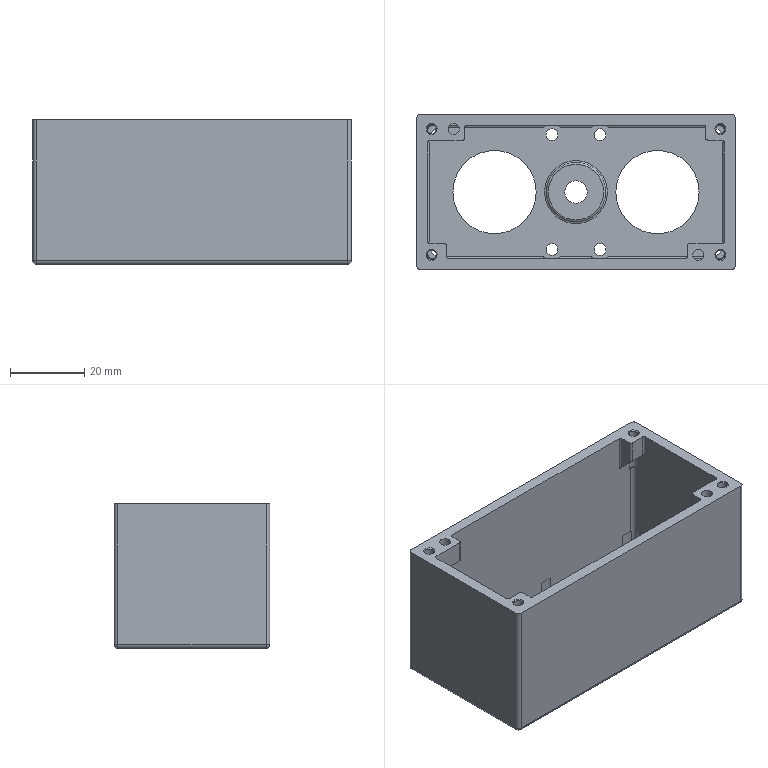Component | NX | DJZ_01_BRACKET_TRAVEL10 | 1 solid | 119 faces | volume 33947 mm3 | cylinder 59 | plane 39 | cone 11 | sphere 4 | spline 4 | torus 2 | commonest cylinder face diameters 1 x20 2 x12 3.2 x8 6 x8 2.5 x4 22.5 x2 3 x2 16 x1